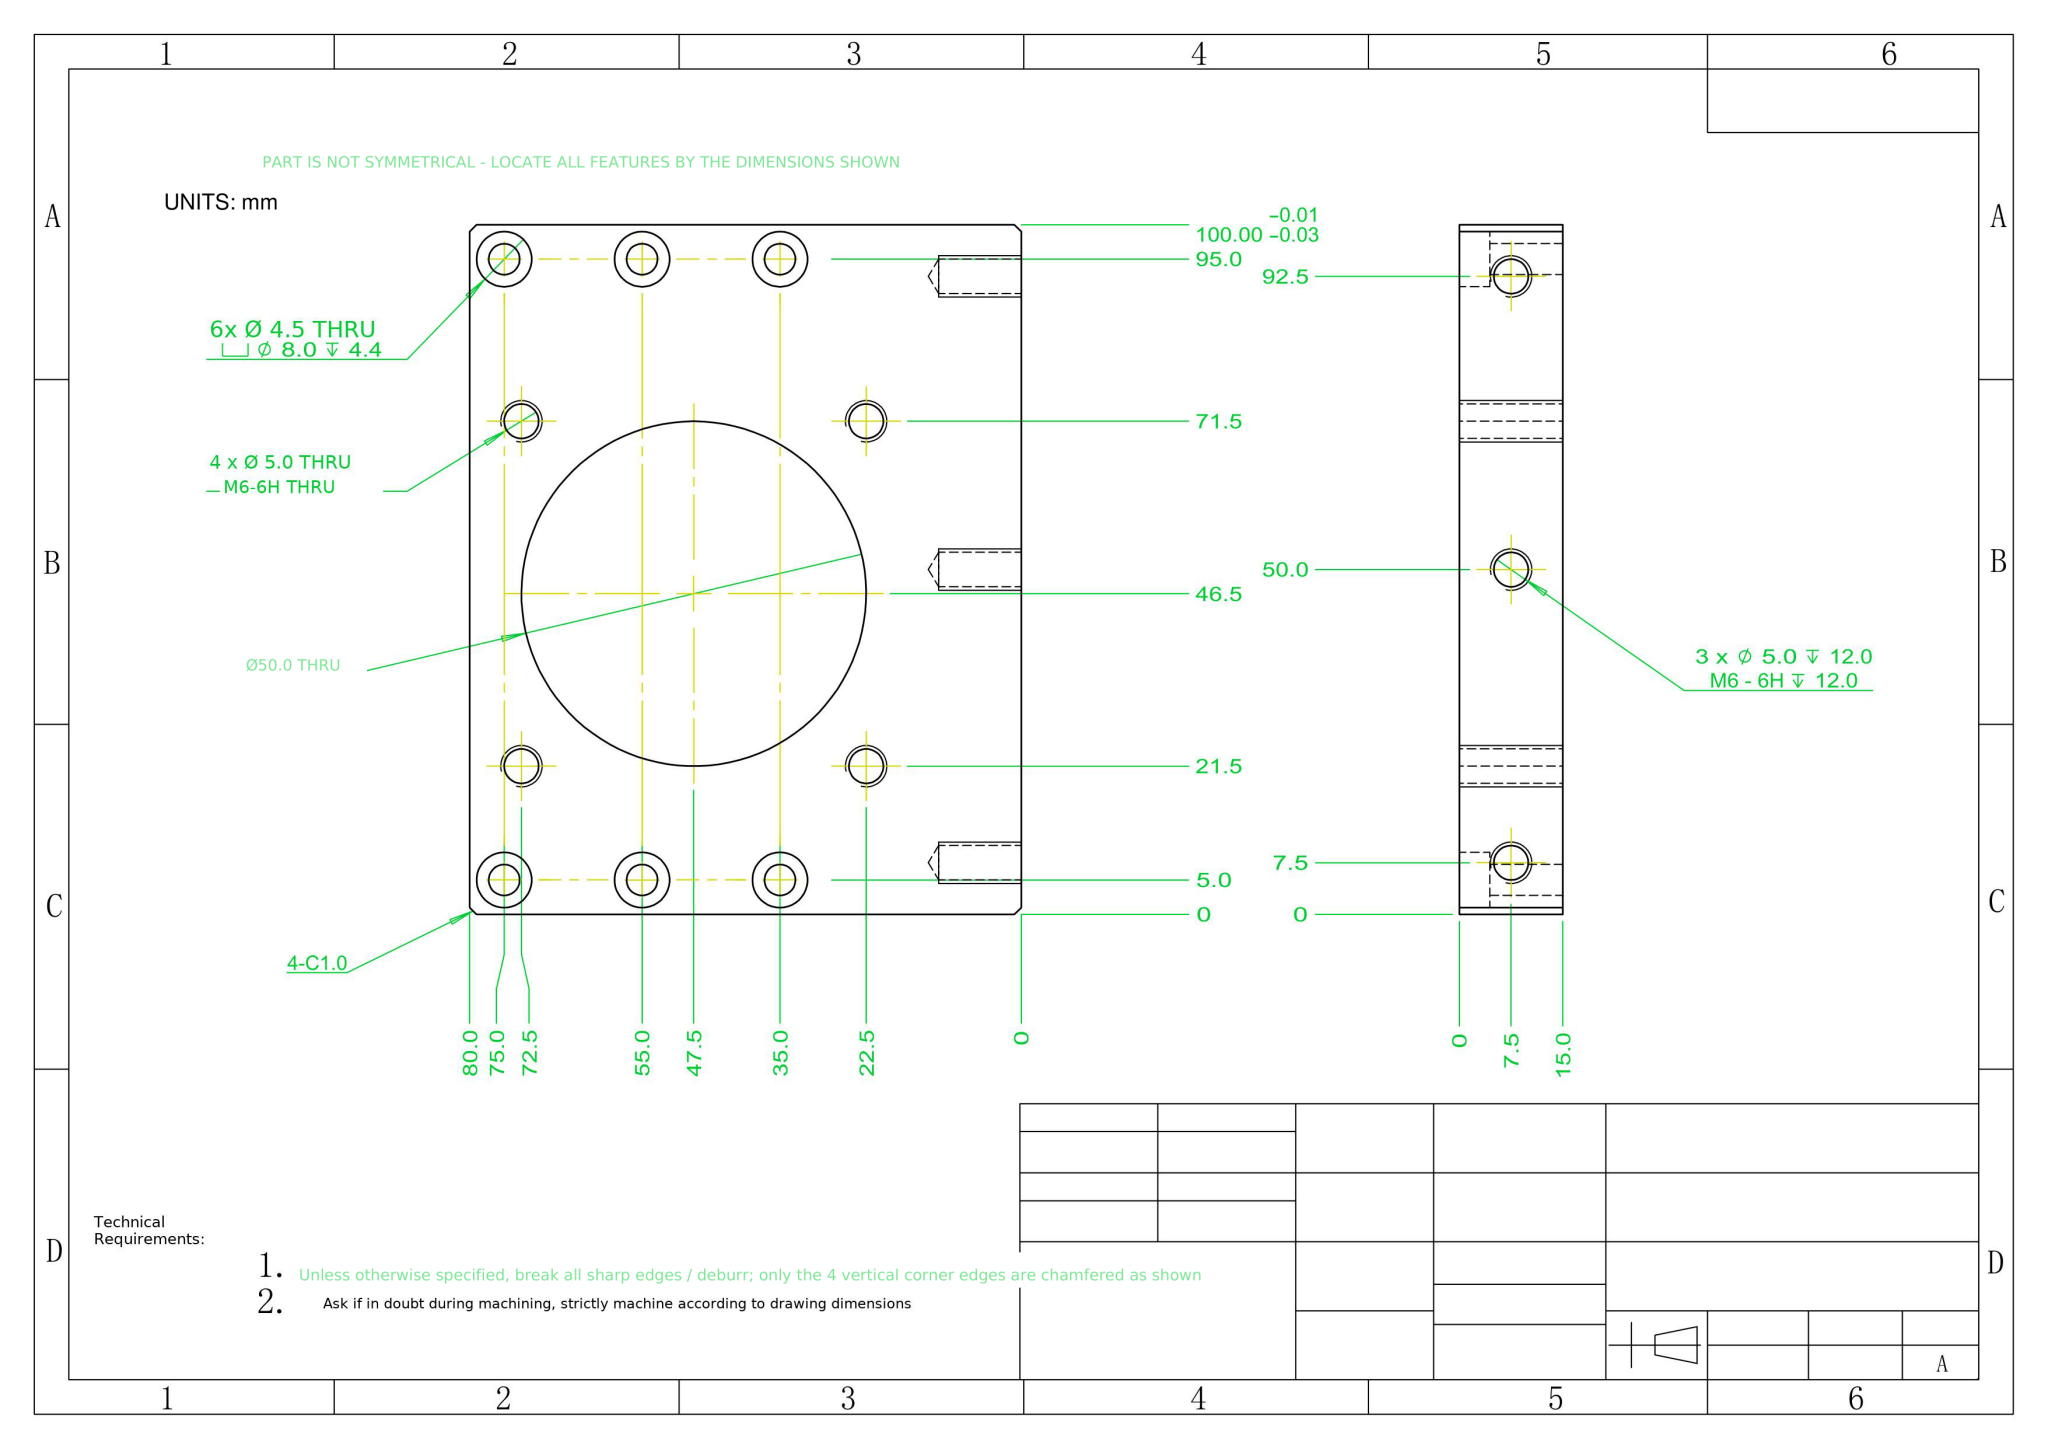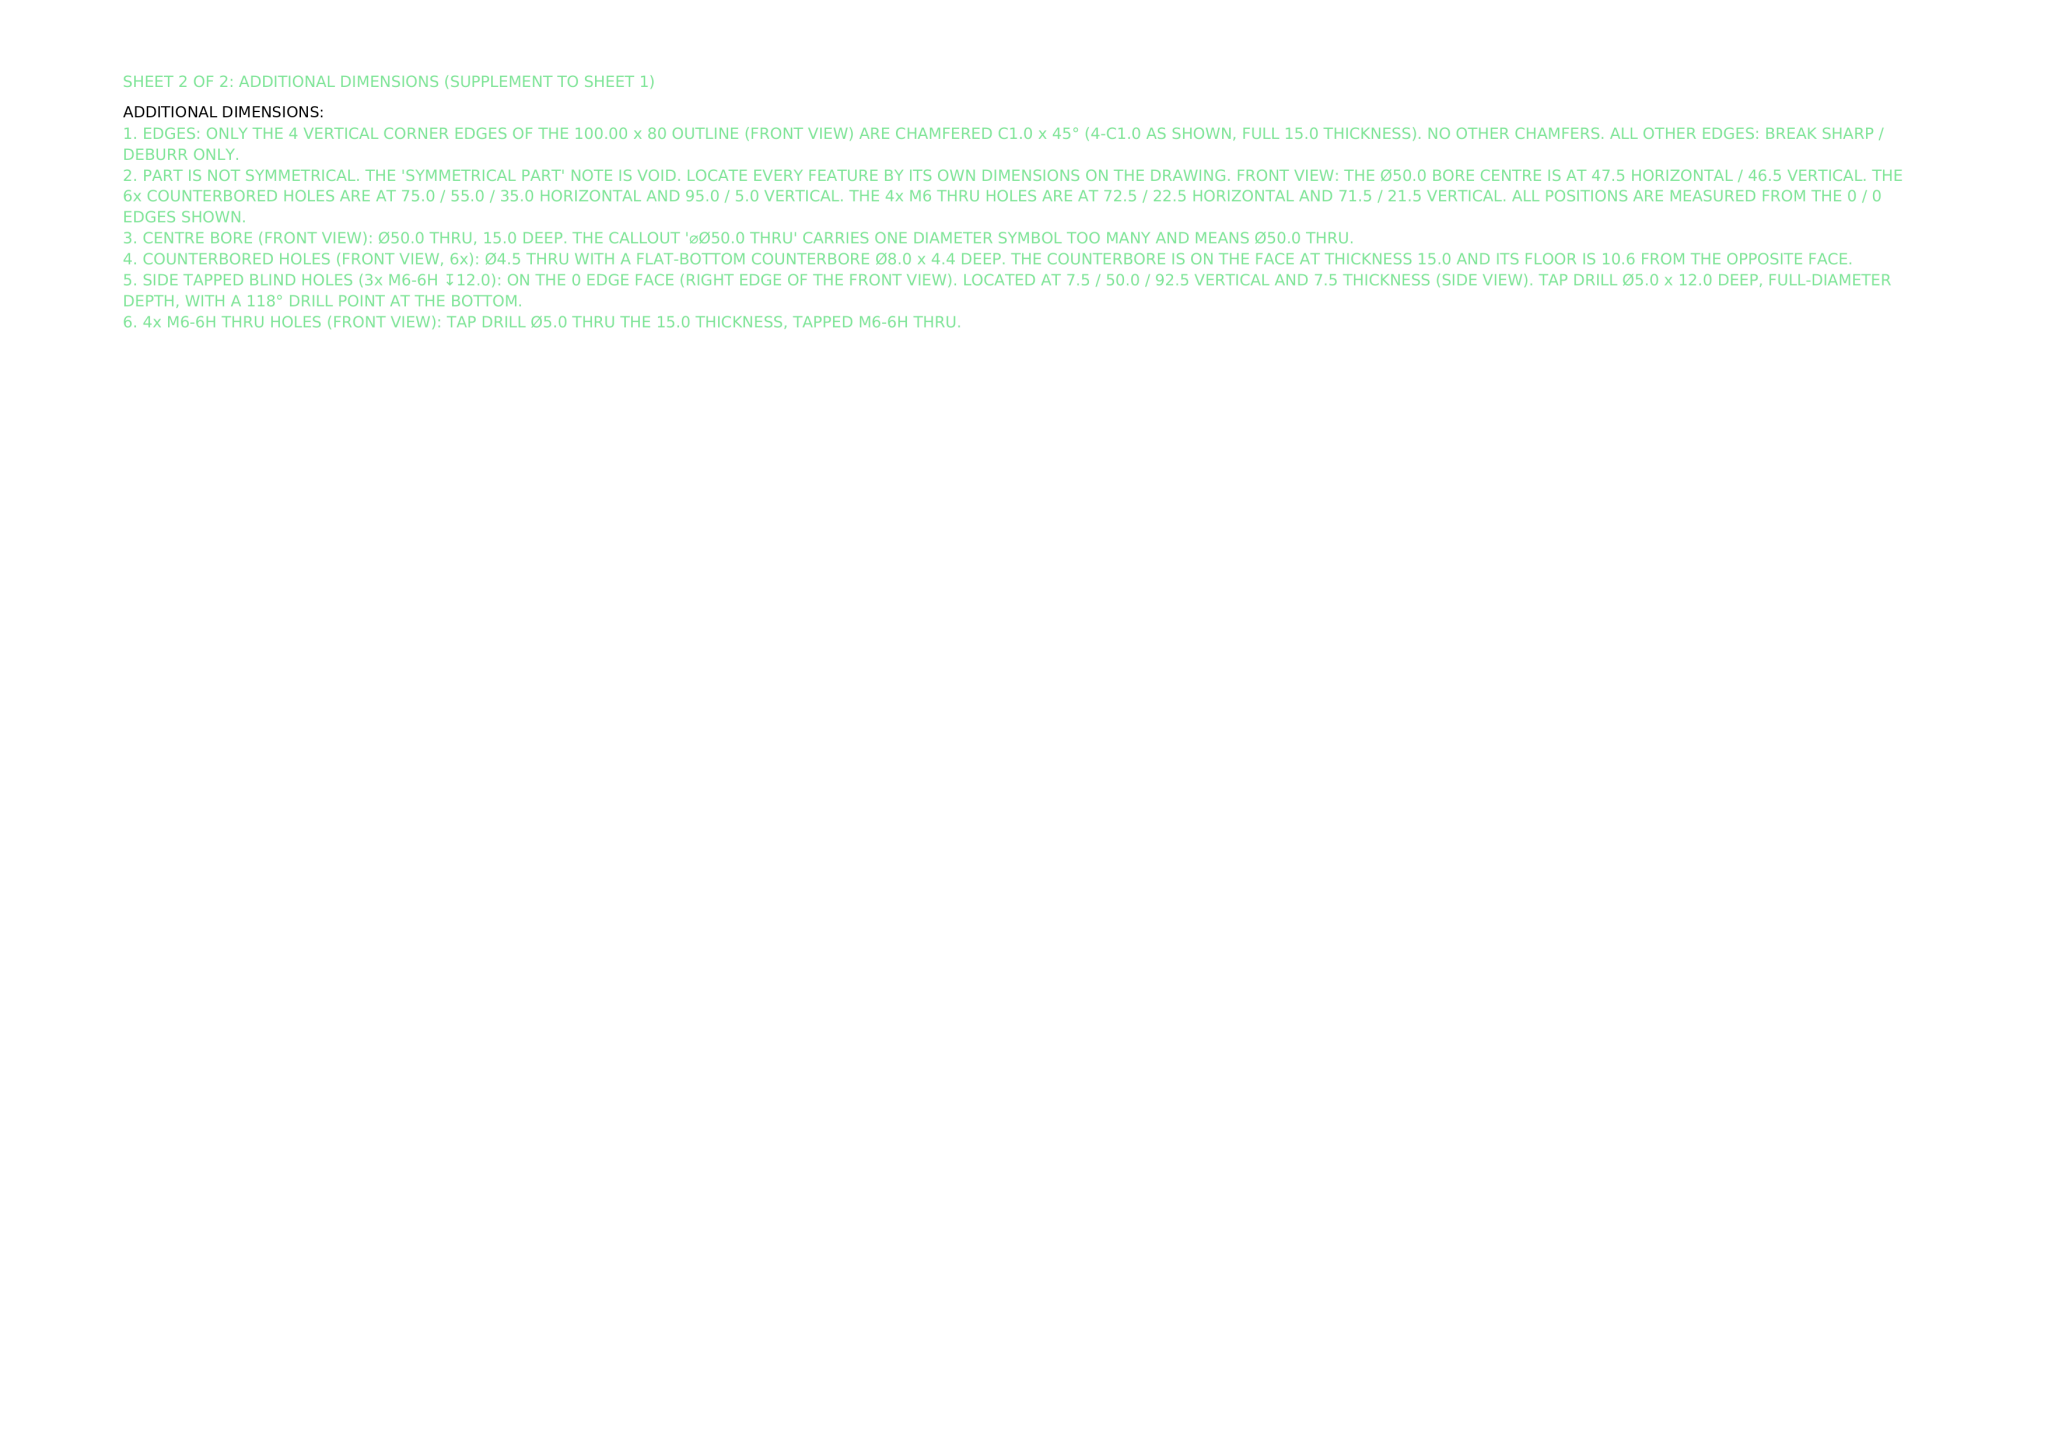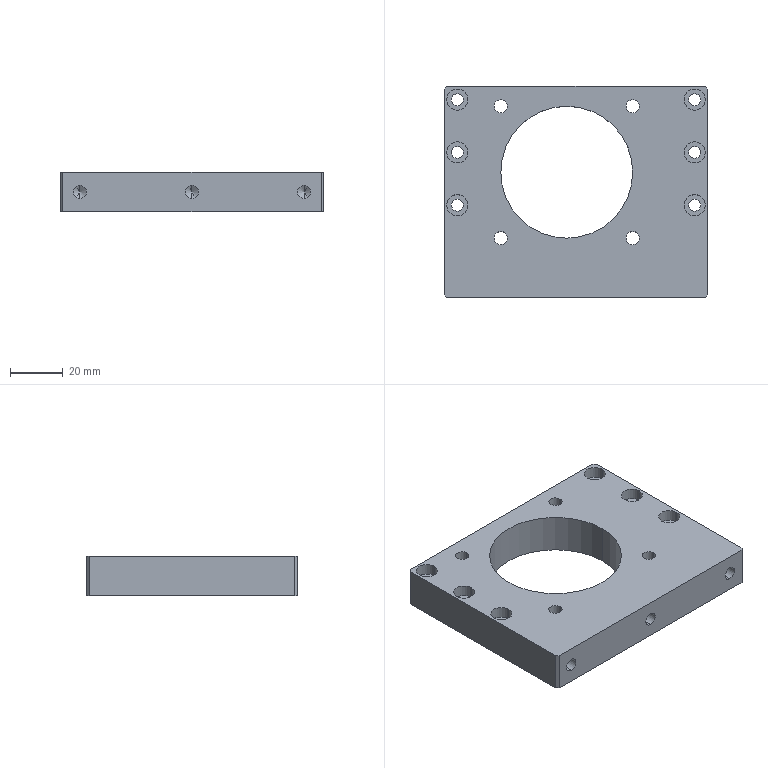Part | NX | mm | 1 solid | 62 faces | box 100 x 80 x 15 mm | volume 86265 mm3 | cylinder 40 | plane 16 | cone 6 | commonest cylinder face diameters 5 x14 8 x12 4.5 x12 50 x2